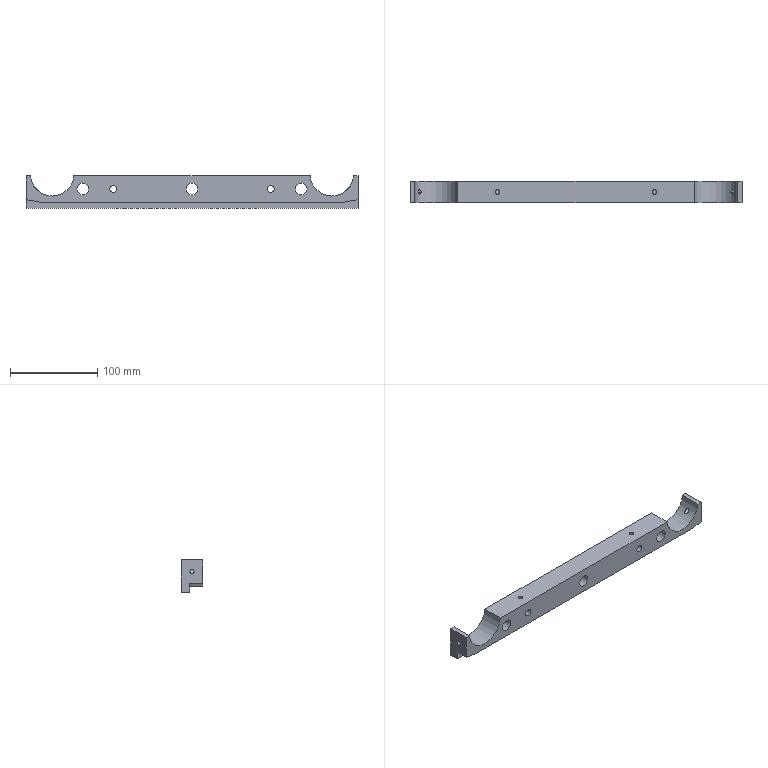Component | SolidWorks | NewDieSet-1_GuideSlot1-01-4 | 1 solid | 41 faces | box 380 x 25.1 x 37 mm | volume 246797 mm3 | cylinder 26 | plane 15 | commonest cylinder face diameters 5 x8 20 x6 13.5 x6 8 x4 50 x2
build123d program:
from build123d import *

# Parameters (mm, degrees)
SKETCH1_W                                            = 30
SKETCH1_H                                            = 380
BOSS_EXTRUDE1_DEPTH                                  = 25.1
SKETCH13_W                                           = 7
SKETCH13_H                                           = 10
BOSS_EXTRUDE2_DEPTH                                  = 380
HOLE_SIZE_ACCORDING_TO_HEXAGON_SOCKET_HE_D           = 13.5
HOLE_SIZE_ACCORDING_TO_HEXAGON_SOCKET_HE_CBORE_D     = 20
HOLE_SIZE_ACCORDING_TO_HEXAGON_SOCKET_HE_CBORE_DEPTH = 13
SKETCH5_R                                            = 4
CUT_EXTRUDE5_DEPTH                                   = 132
SKETCH20_R                                           = 25
CUT_EXTRUDE12_DEPTH                                  = 383.008
CHAMFER3_SIZE                                        = 15
CHAMFER3_SIZE2                                       = 2.645
M6_TAPPED_HOLE2_D                                    = 5
M6_TAPPED_HOLE2_DEPTH                                = 15
M6_TAPPED_HOLE2_TIP                                  = 1.502


with BuildPart() as part:
    # Sketch1 → Boss-Extrude1 (new body)
    with BuildSketch(Plane(origin=(0, 0, 0), x_dir=(1, 0, 0), z_dir=(0, 1, 0))):
        with Locations((-15, 190)):
            Rectangle(SKETCH1_W, SKETCH1_H)
    extrude(amount=BOSS_EXTRUDE1_DEPTH)

    # Sketch13 → Boss-Extrude2 (add)
    with BuildSketch(Plane(origin=(0, 0, -380), x_dir=(-1, 0, 0), z_dir=(0, 0, -1))):
        with Locations((-3.5, 20.1)):
            Rectangle(SKETCH13_W, SKETCH13_H)
    extrude(amount=-BOSS_EXTRUDE2_DEPTH)

    # Hole Size_According to_Hexagon Socket He (through all)
    with Locations(Plane(origin=(0, 25.1, 0), x_dir=(1, 0, 0), z_dir=(0, 1, 0))):
        with Locations((-15, 315), (-15, 65), (-15, 190)):
            CounterBoreHole(HOLE_SIZE_ACCORDING_TO_HEXAGON_SOCKET_HE_D / 2, HOLE_SIZE_ACCORDING_TO_HEXAGON_SOCKET_HE_CBORE_D / 2, HOLE_SIZE_ACCORDING_TO_HEXAGON_SOCKET_HE_CBORE_DEPTH)

    # Sketch5 → Cut-Extrude5 (cut)
    with BuildSketch(Plane.XZ):
        with Locations(Location((-15, -100, 0), (0, 0, 270))):
            Circle(SKETCH5_R)
        with Locations(Location((-15, -280, 0), (0, 0, 270))):
            Circle(SKETCH5_R)
    extrude(amount=-CUT_EXTRUDE5_DEPTH, mode=Mode.SUBTRACT)

    # Sketch20 → Cut-Extrude12 (cut, through all)
    with BuildSketch(Plane(origin=(0, 25.1, 0), x_dir=(1, 0, 0), z_dir=(0, 1, 0))):
        with Locations((-31.9, 30)):
            Circle(SKETCH20_R)
    cut_extrude12 = extrude(amount=-CUT_EXTRUDE12_DEPTH, mode=Mode.SUBTRACT)

    # Mirror2: Cut-Extrude12 across plane
    add(cut_extrude12.mirror(Plane(origin=(0, 0, -190), x_dir=(1, 0, 0), z_dir=(0, 0, -1))), mode=Mode.SUBTRACT)

    # Chamfer3
    chamfer3_edges = [part.edges().sort_by_distance(p)[0] for p in [
        (0, 7.55, 0),
        (0, 7.55, -380),
    ]]
    chamfer3_side = [part.faces().sort_by_distance(p)[0] for p in [
        (0, 7.55, -190),
    ]]
    chamfer(chamfer3_edges, length=CHAMFER3_SIZE, length2=CHAMFER3_SIZE2, reference=chamfer3_side[0])

    # Sketch21 → M6 Tapped Hole1 (revolve, cut)
    with BuildSketch(Plane(origin=(-16.322, 12.55, -380), x_dir=(0, 1, 0), z_dir=(1, 0, 0))):
        Polygon((0, 0), (0, 24.502), (2.5, 23), (2.5, 0), align=None)
    m6_tapped_hole1 = revolve(axis=Axis((-16.322, 12.55, -386.35), (0, 0, 1)), mode=Mode.SUBTRACT)

    # Mirror3: M6 Tapped Hole1 across plane
    add(m6_tapped_hole1.mirror(Plane(origin=(0, 0, -190), x_dir=(1, 0, 0), z_dir=(0, 0, -1))), mode=Mode.SUBTRACT)

    # M6 Tapped Hole2
    with Locations(Plane.ZY.offset(30)):
        with Locations((-280, 12.55), (-100, 12.55)):
            Hole(M6_TAPPED_HOLE2_D / 2, depth=M6_TAPPED_HOLE2_DEPTH)
            with Locations((0, 0, -(M6_TAPPED_HOLE2_DEPTH + M6_TAPPED_HOLE2_TIP / 2))):  # 118° drill point
                Cone(0, M6_TAPPED_HOLE2_D / 2, M6_TAPPED_HOLE2_TIP, mode=Mode.SUBTRACT)


solid = part.part

# Placed as in the assembly
solid = solid.moved(Location((133.254, 5.927, 536.1), (0, 90, 0)))